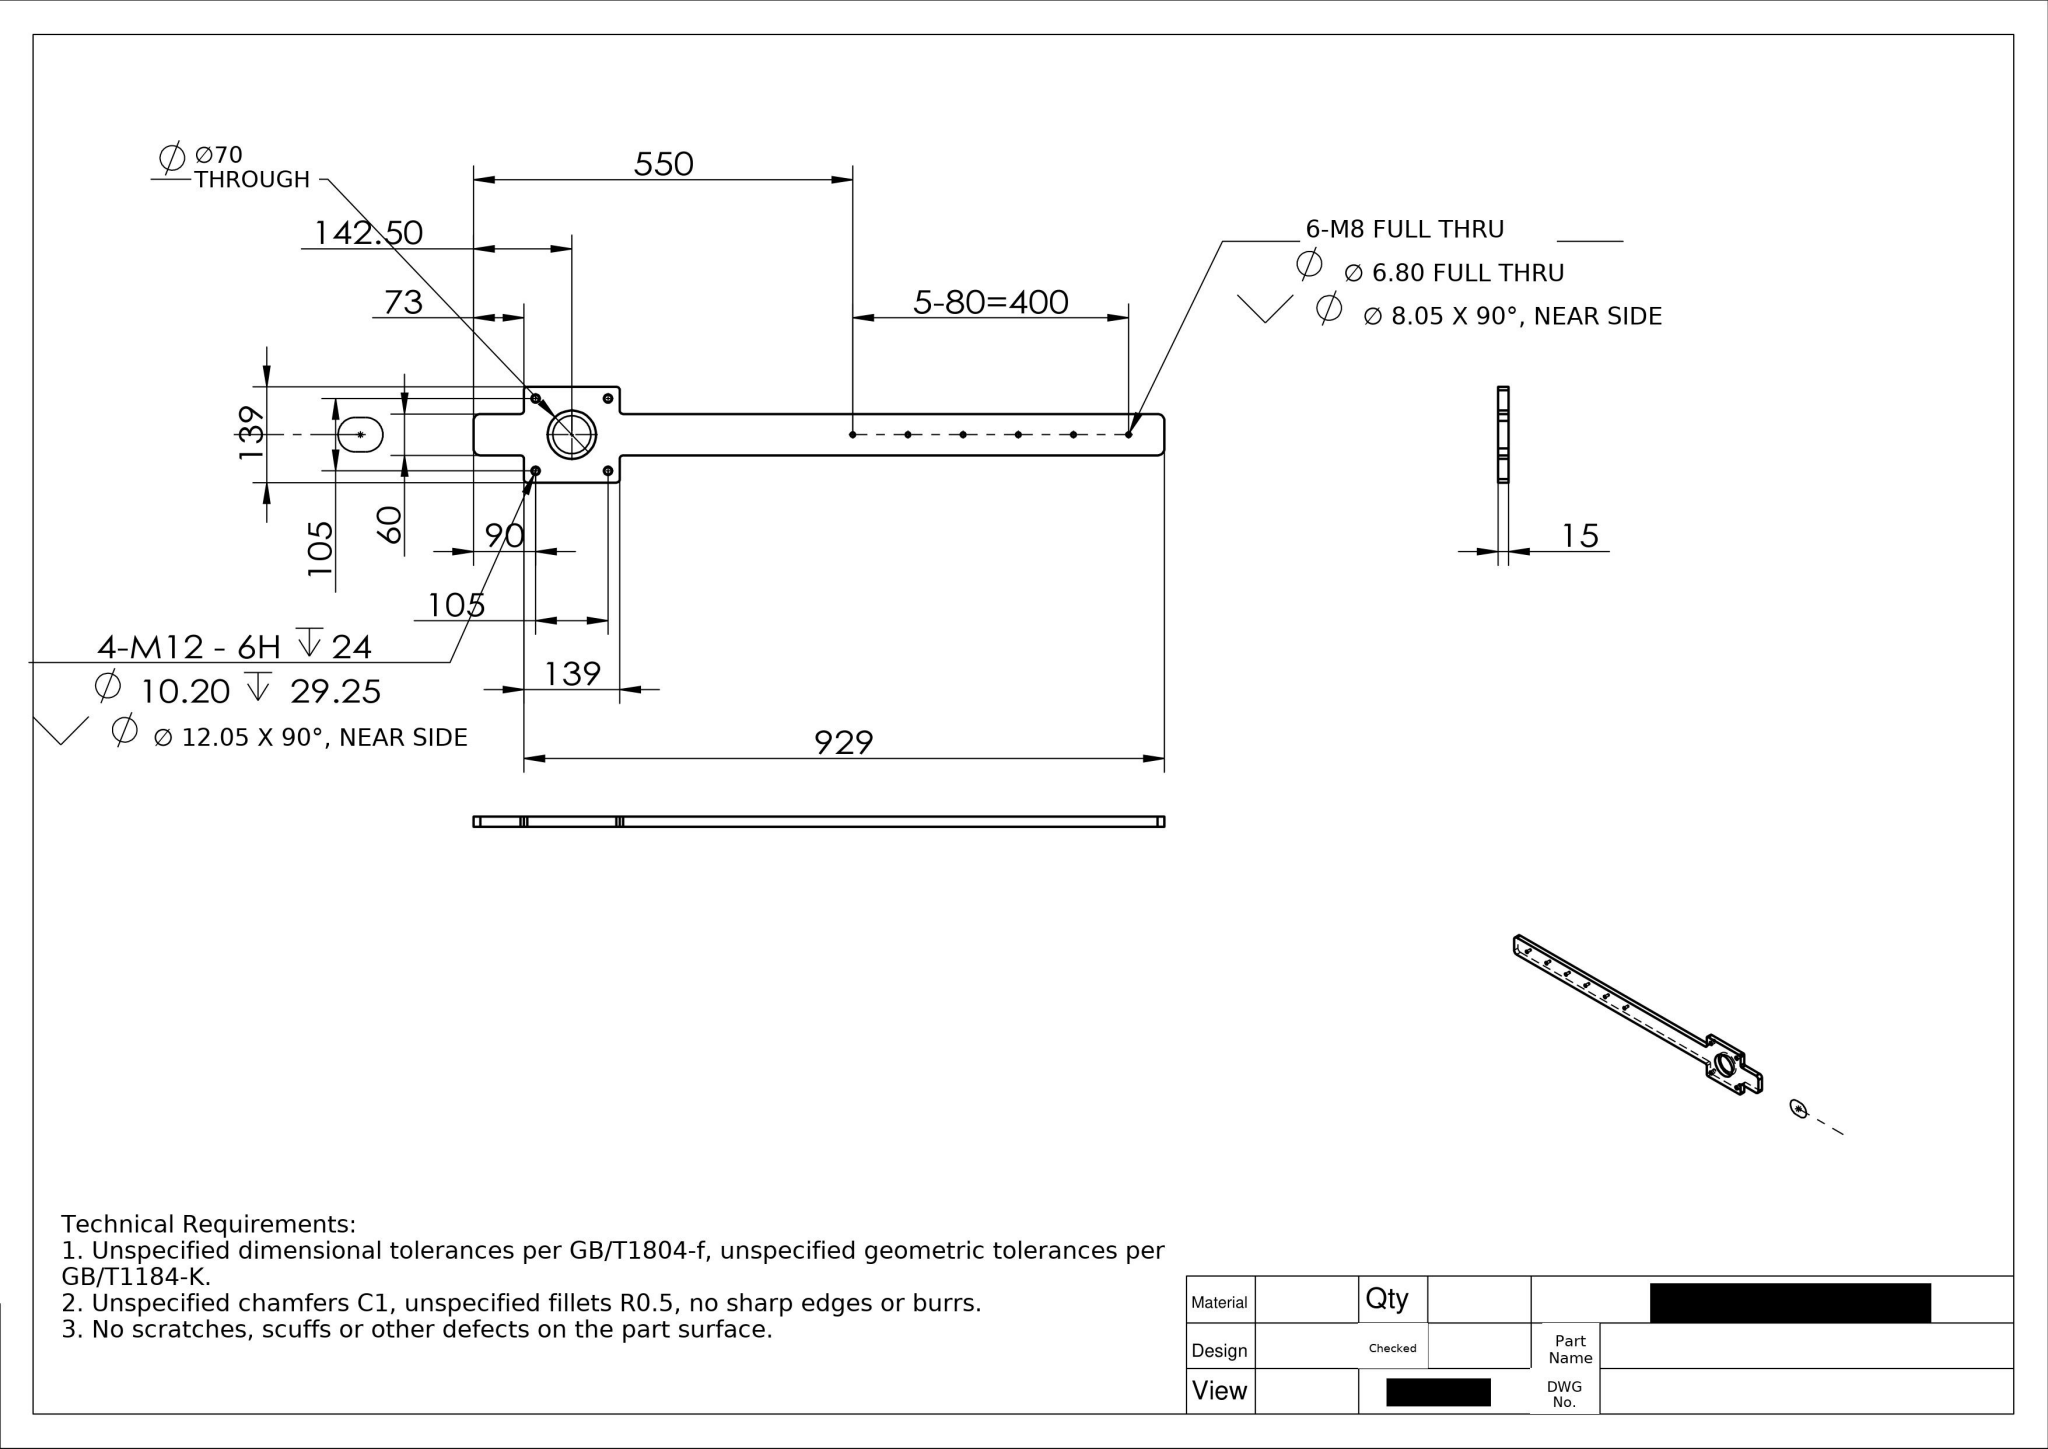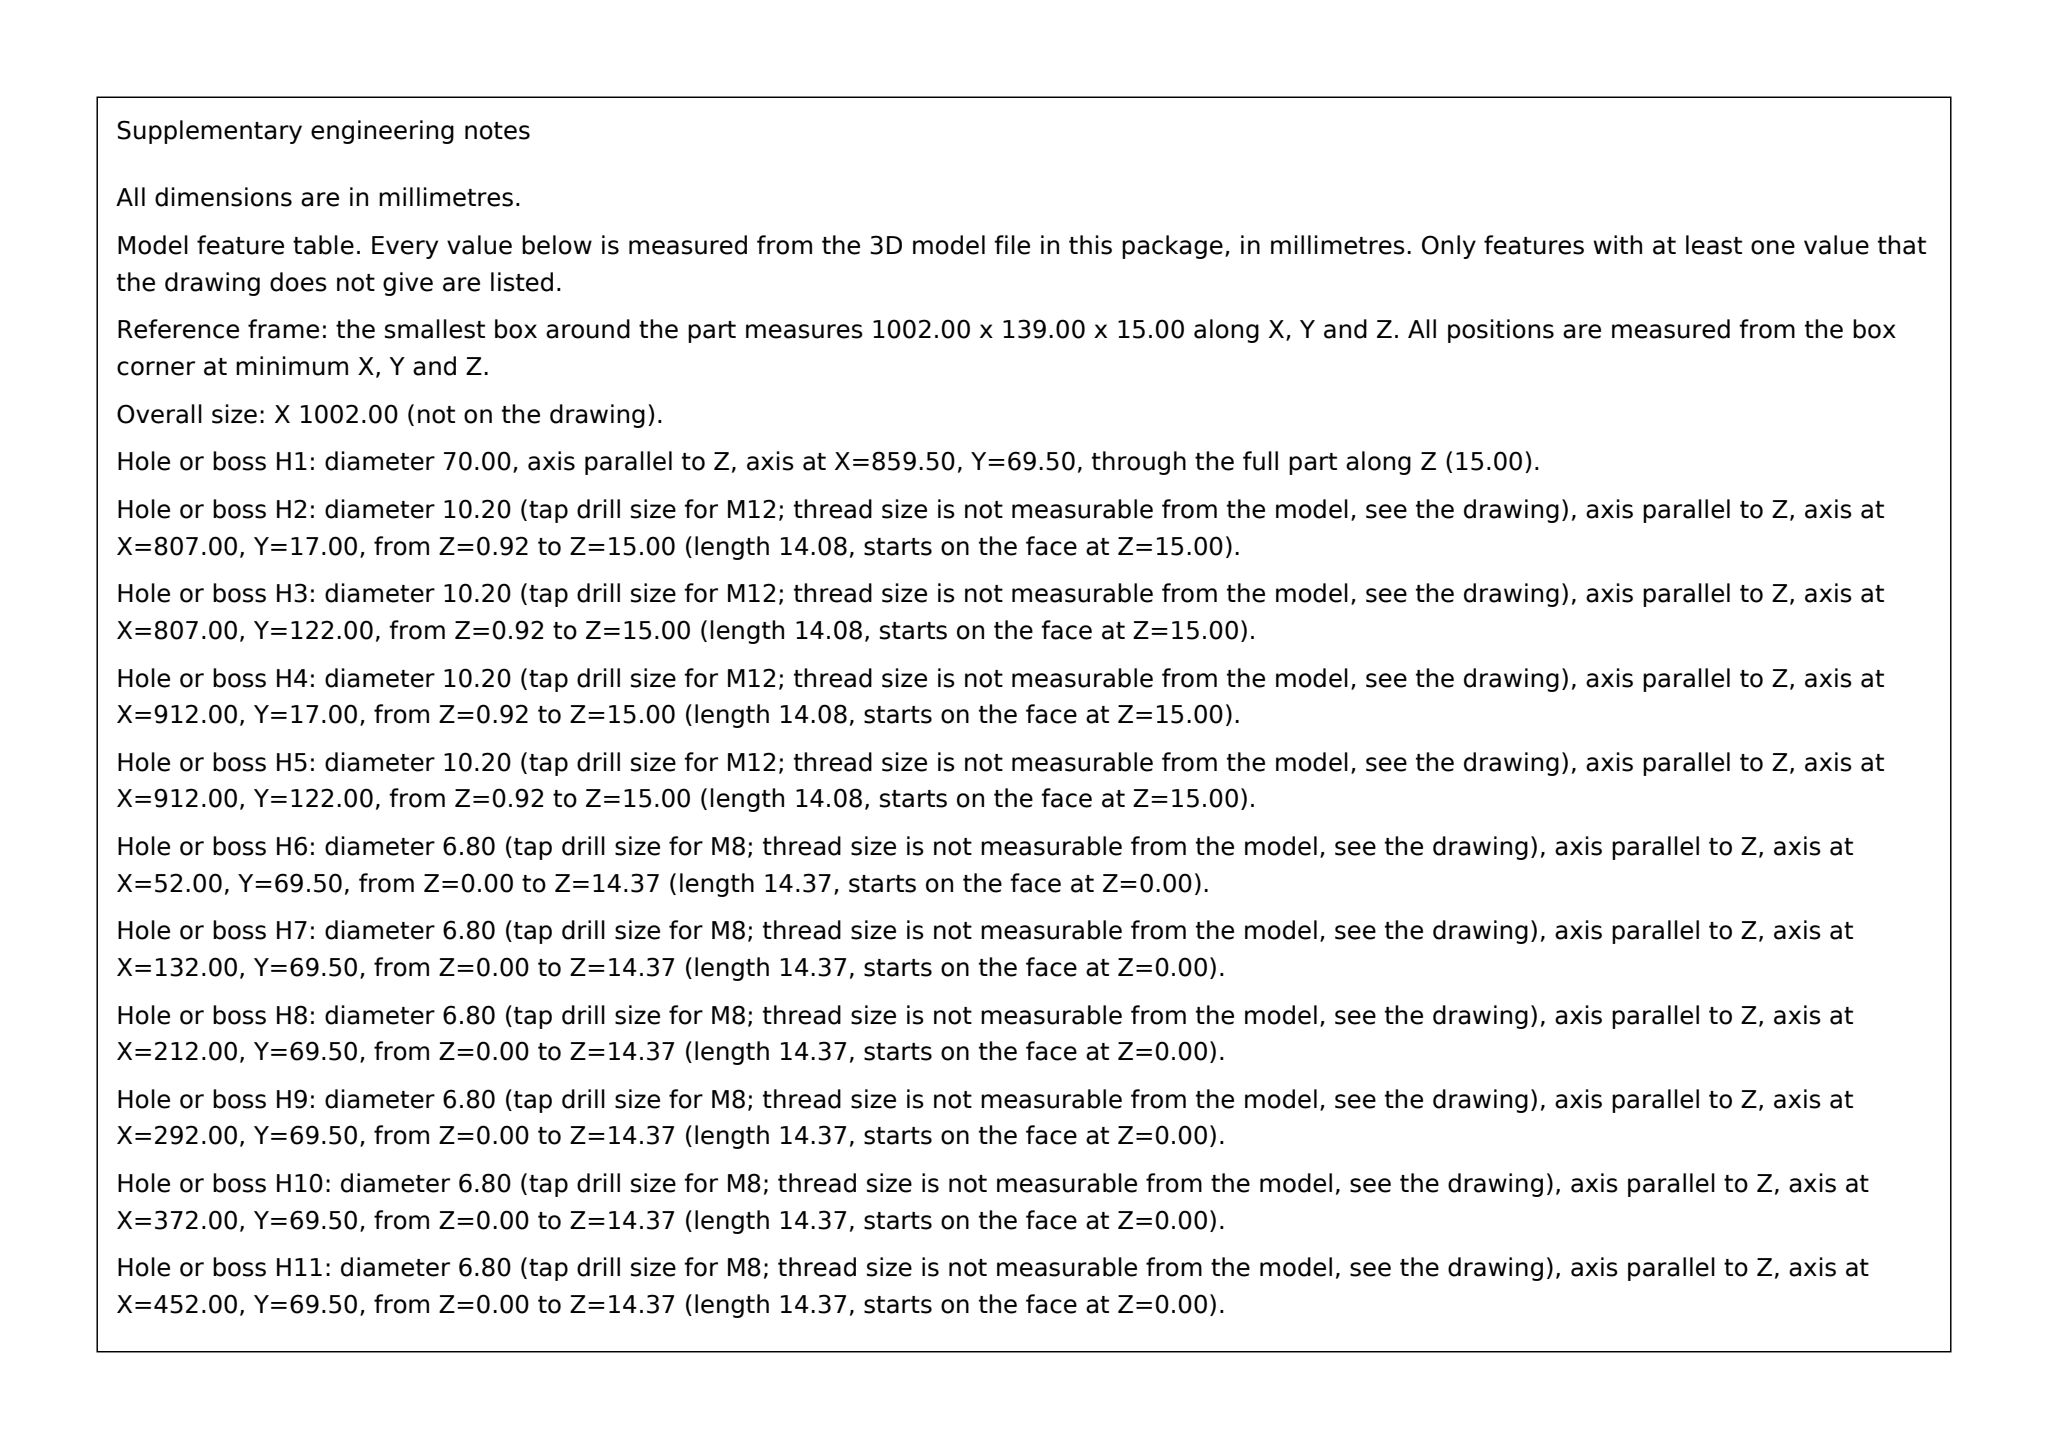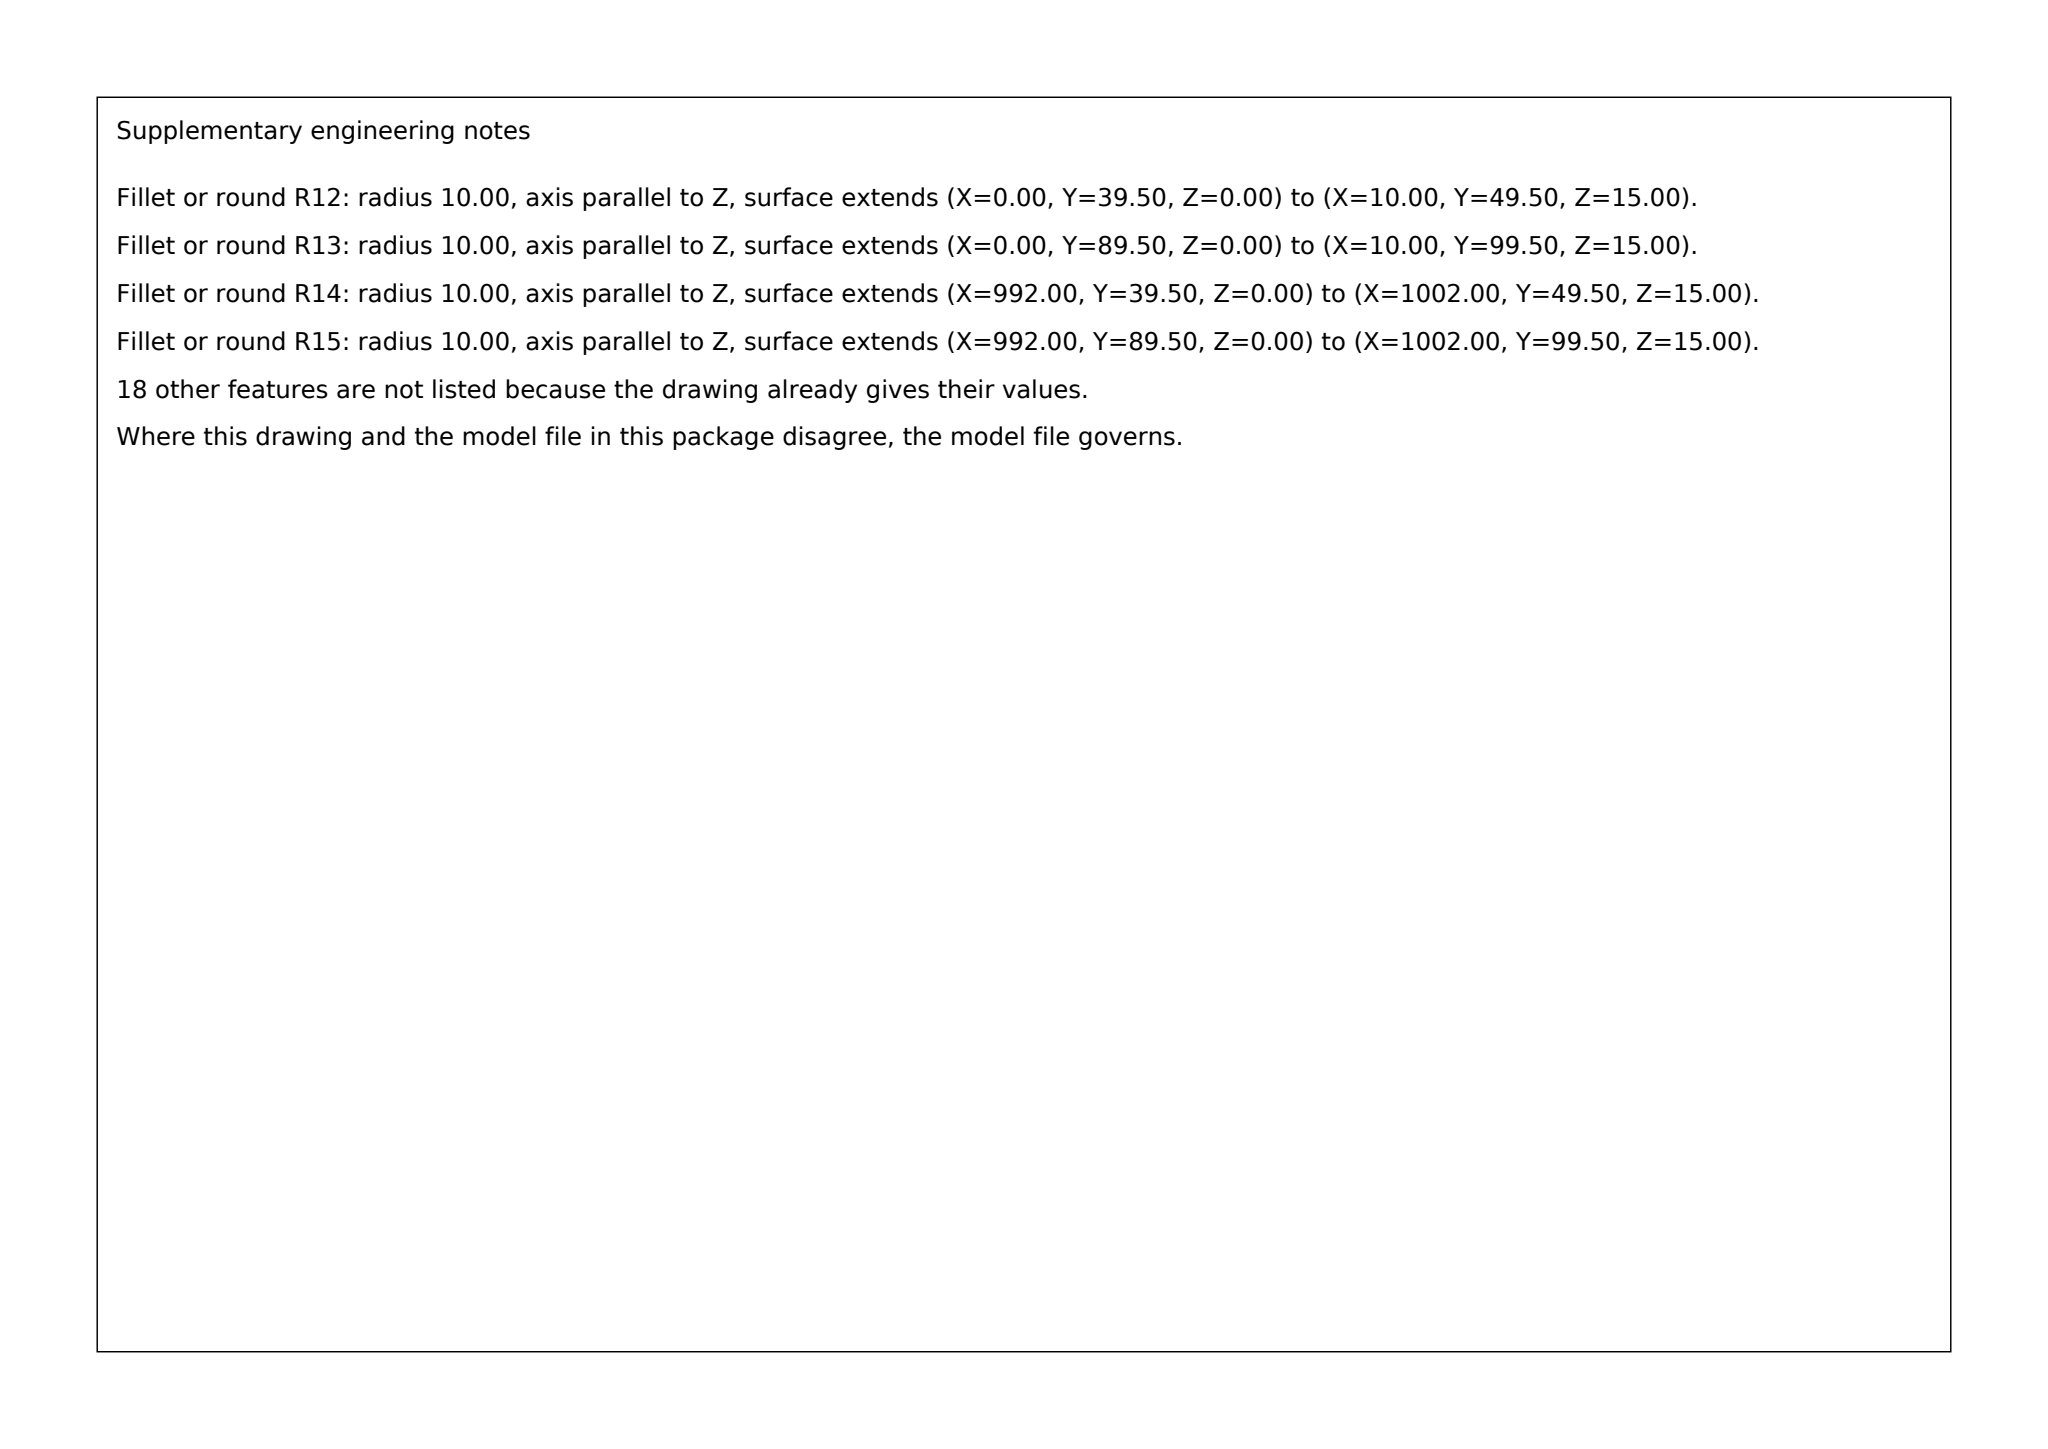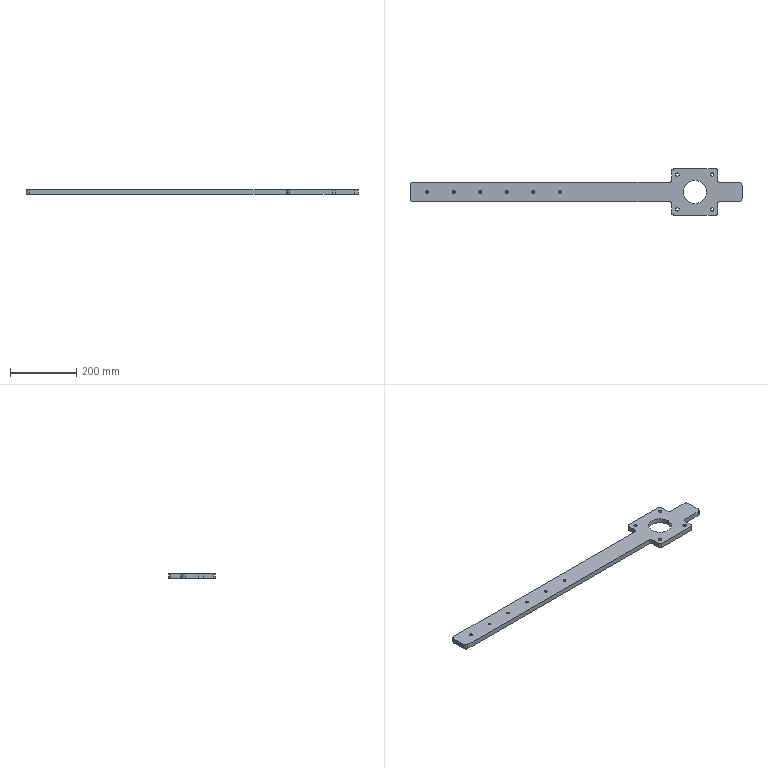Part | SolidWorks | mm | 1 solid | 68 faces | box 1002 x 139 x 15 mm | volume 999245 mm3 | cylinder 34 | cone 20 | plane 14 | commonest cylinder face diameters 6.8 x12 10.2 x8 10 x8 20 x4 70 x2
build123d program:
from build123d import *

# Parameters (mm, degrees)
SKETCH1_W                    = 1002
SKETCH1_H                    = 60
BOSS_EXTRUDE1_DEPTH          = 15
FILLET1_R                    = 10
M8_TAPPED_HOLE1_D            = 6.8
M8_TAPPED_HOLE1_CSINK_D      = 8.05
M8_TAPPED_HOLE1_CSINK_ANGLE  = 90
SKETCH8_W                    = 139
SKETCH8_H                    = 39.5
BOSS_EXTRUDE2_DEPTH          = 15
M12_TAPPED_HOLE1_D           = 10.2
M12_TAPPED_HOLE1_DEPTH       = 29.25
M12_TAPPED_HOLE1_CSINK_D     = 12.05
M12_TAPPED_HOLE1_CSINK_ANGLE = 90
M12_TAPPED_HOLE1_TIP         = 3.064
SKETCH6_R                    = 35
CUT_EXTRUDE1_DEPTH           = 507.02
FILLET2_R                    = 5


with BuildPart() as part:
    # Sketch1 → Boss-Extrude1 (new body)
    with BuildSketch(Plane.XY):
        Rectangle(SKETCH1_W, SKETCH1_H)
    extrude(amount=BOSS_EXTRUDE1_DEPTH)

    # Fillet1
    fillet1_edges = [part.edges().sort_by_distance(p)[0] for p in [
        (-501, 30, 7.5),
        (501, 30, 7.5),
        (501, -30, 7.5),
        (-501, -30, 7.5),
    ]]
    fillet(fillet1_edges, radius=FILLET1_R)

    # M8 Tapped Hole1 (through all)
    with Locations(Plane.XY.offset(15)):
        with Locations((-49, 0), (-129, 0), (-209, 0), (-289, 0), (-369, 0), (-449, 0), (-529, 0), (-769, 0), (-689, 0), (-609, 0)):
            CounterSinkHole(M8_TAPPED_HOLE1_D / 2, M8_TAPPED_HOLE1_CSINK_D / 2, counter_sink_angle=M8_TAPPED_HOLE1_CSINK_ANGLE)

    # Sketch8 → Boss-Extrude2 (add)
    with BuildSketch(Plane.XY.offset(15)):
        with Locations((358.5, -49.75)):
            Rectangle(SKETCH8_W, SKETCH8_H)
        with Locations((358.5, 49.75)):
            Rectangle(SKETCH8_W, SKETCH8_H)
    extrude(amount=-BOSS_EXTRUDE2_DEPTH)

    # M12 Tapped Hole1
    with Locations(Plane(origin=(0, 0, 0), x_dir=(-1, 0, 0), z_dir=(0, 0, -1))):
        with Locations((-306, -52.5), (-411, -52.5), (-411, 52.5), (-306, 52.5)):
            CounterSinkHole(M12_TAPPED_HOLE1_D / 2, M12_TAPPED_HOLE1_CSINK_D / 2, depth=M12_TAPPED_HOLE1_DEPTH, counter_sink_angle=M12_TAPPED_HOLE1_CSINK_ANGLE)
            with Locations((0, 0, -(M12_TAPPED_HOLE1_DEPTH + M12_TAPPED_HOLE1_TIP / 2))):  # 118° drill point
                Cone(0, M12_TAPPED_HOLE1_D / 2, M12_TAPPED_HOLE1_TIP, mode=Mode.SUBTRACT)

    # Sketch6 → Cut-Extrude1 (cut, through all)
    with BuildSketch(Plane(origin=(0, 0, 0), x_dir=(-1, 0, 0), z_dir=(0, 0, -1))):
        with Locations((-358.5, 0)):
            Circle(SKETCH6_R)
    extrude(amount=-CUT_EXTRUDE1_DEPTH, mode=Mode.SUBTRACT)

    # Fillet2
    fillet2_edges = [part.edges().sort_by_distance(p)[0] for p in [
        (428, -69.5, 7.5),
        (428, -30, 7.5),
        (289, -30, 7.5),
        (289, -69.5, 7.5),
        (428, 30, 7.5),
        (428, 69.5, 7.5),
        (289, 69.5, 7.5),
        (289, 30, 7.5),
    ]]
    fillet(fillet2_edges, radius=FILLET2_R)


solid = part.part